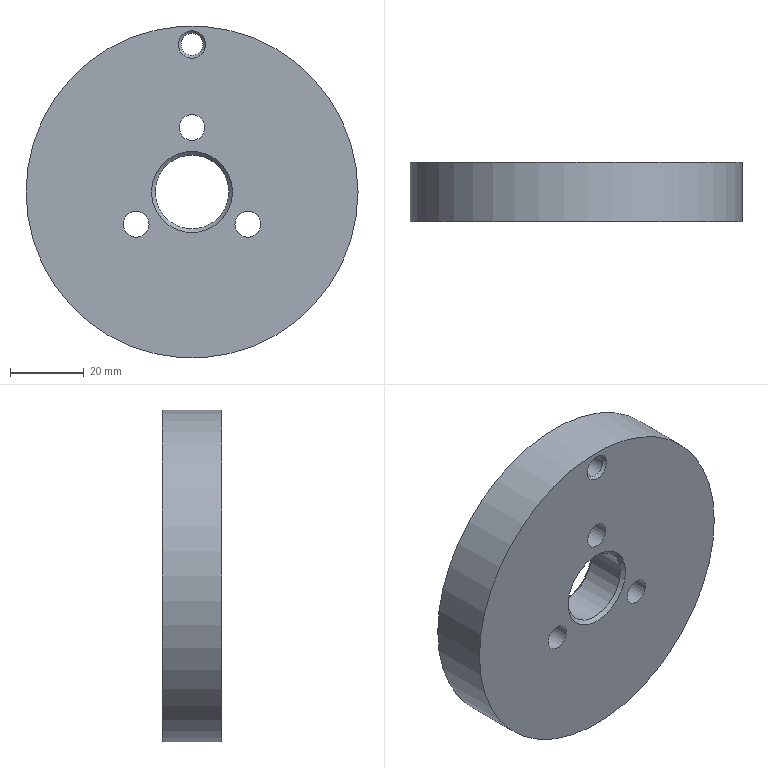Component | NX | 10_HANDWHEEL | 1 solid | 22 faces | volume 75888 mm3 | cylinder 10 | plane 7 | cone 4 | torus 1 | commonest cylinder face diameters 7 x3 11 x3 64 x1 90 x1 20 x1 6 x1